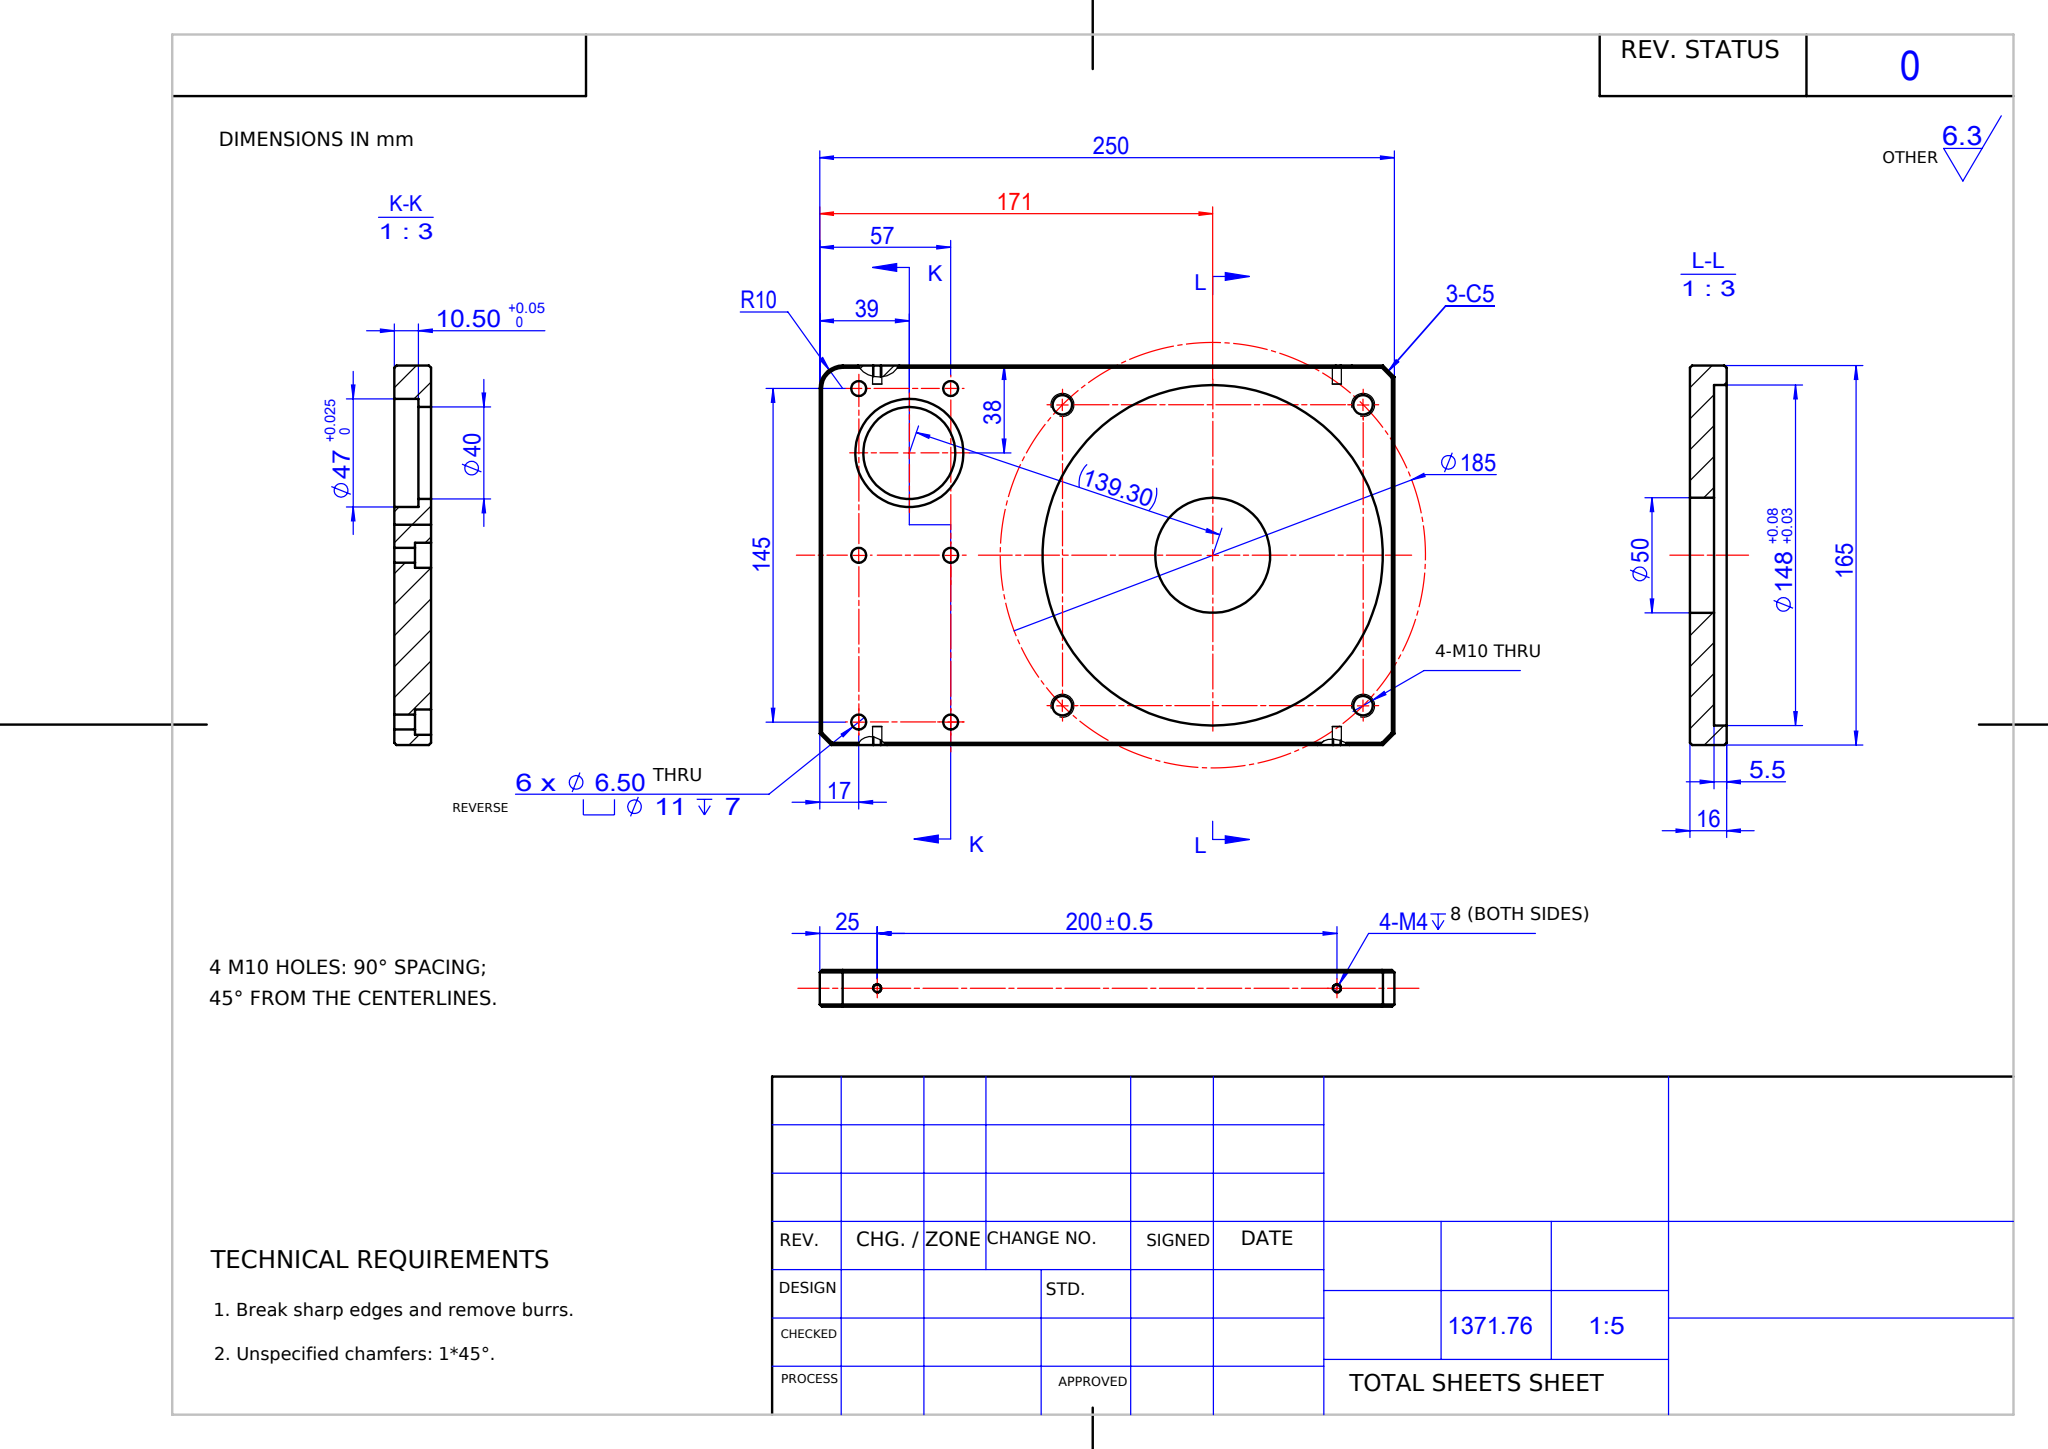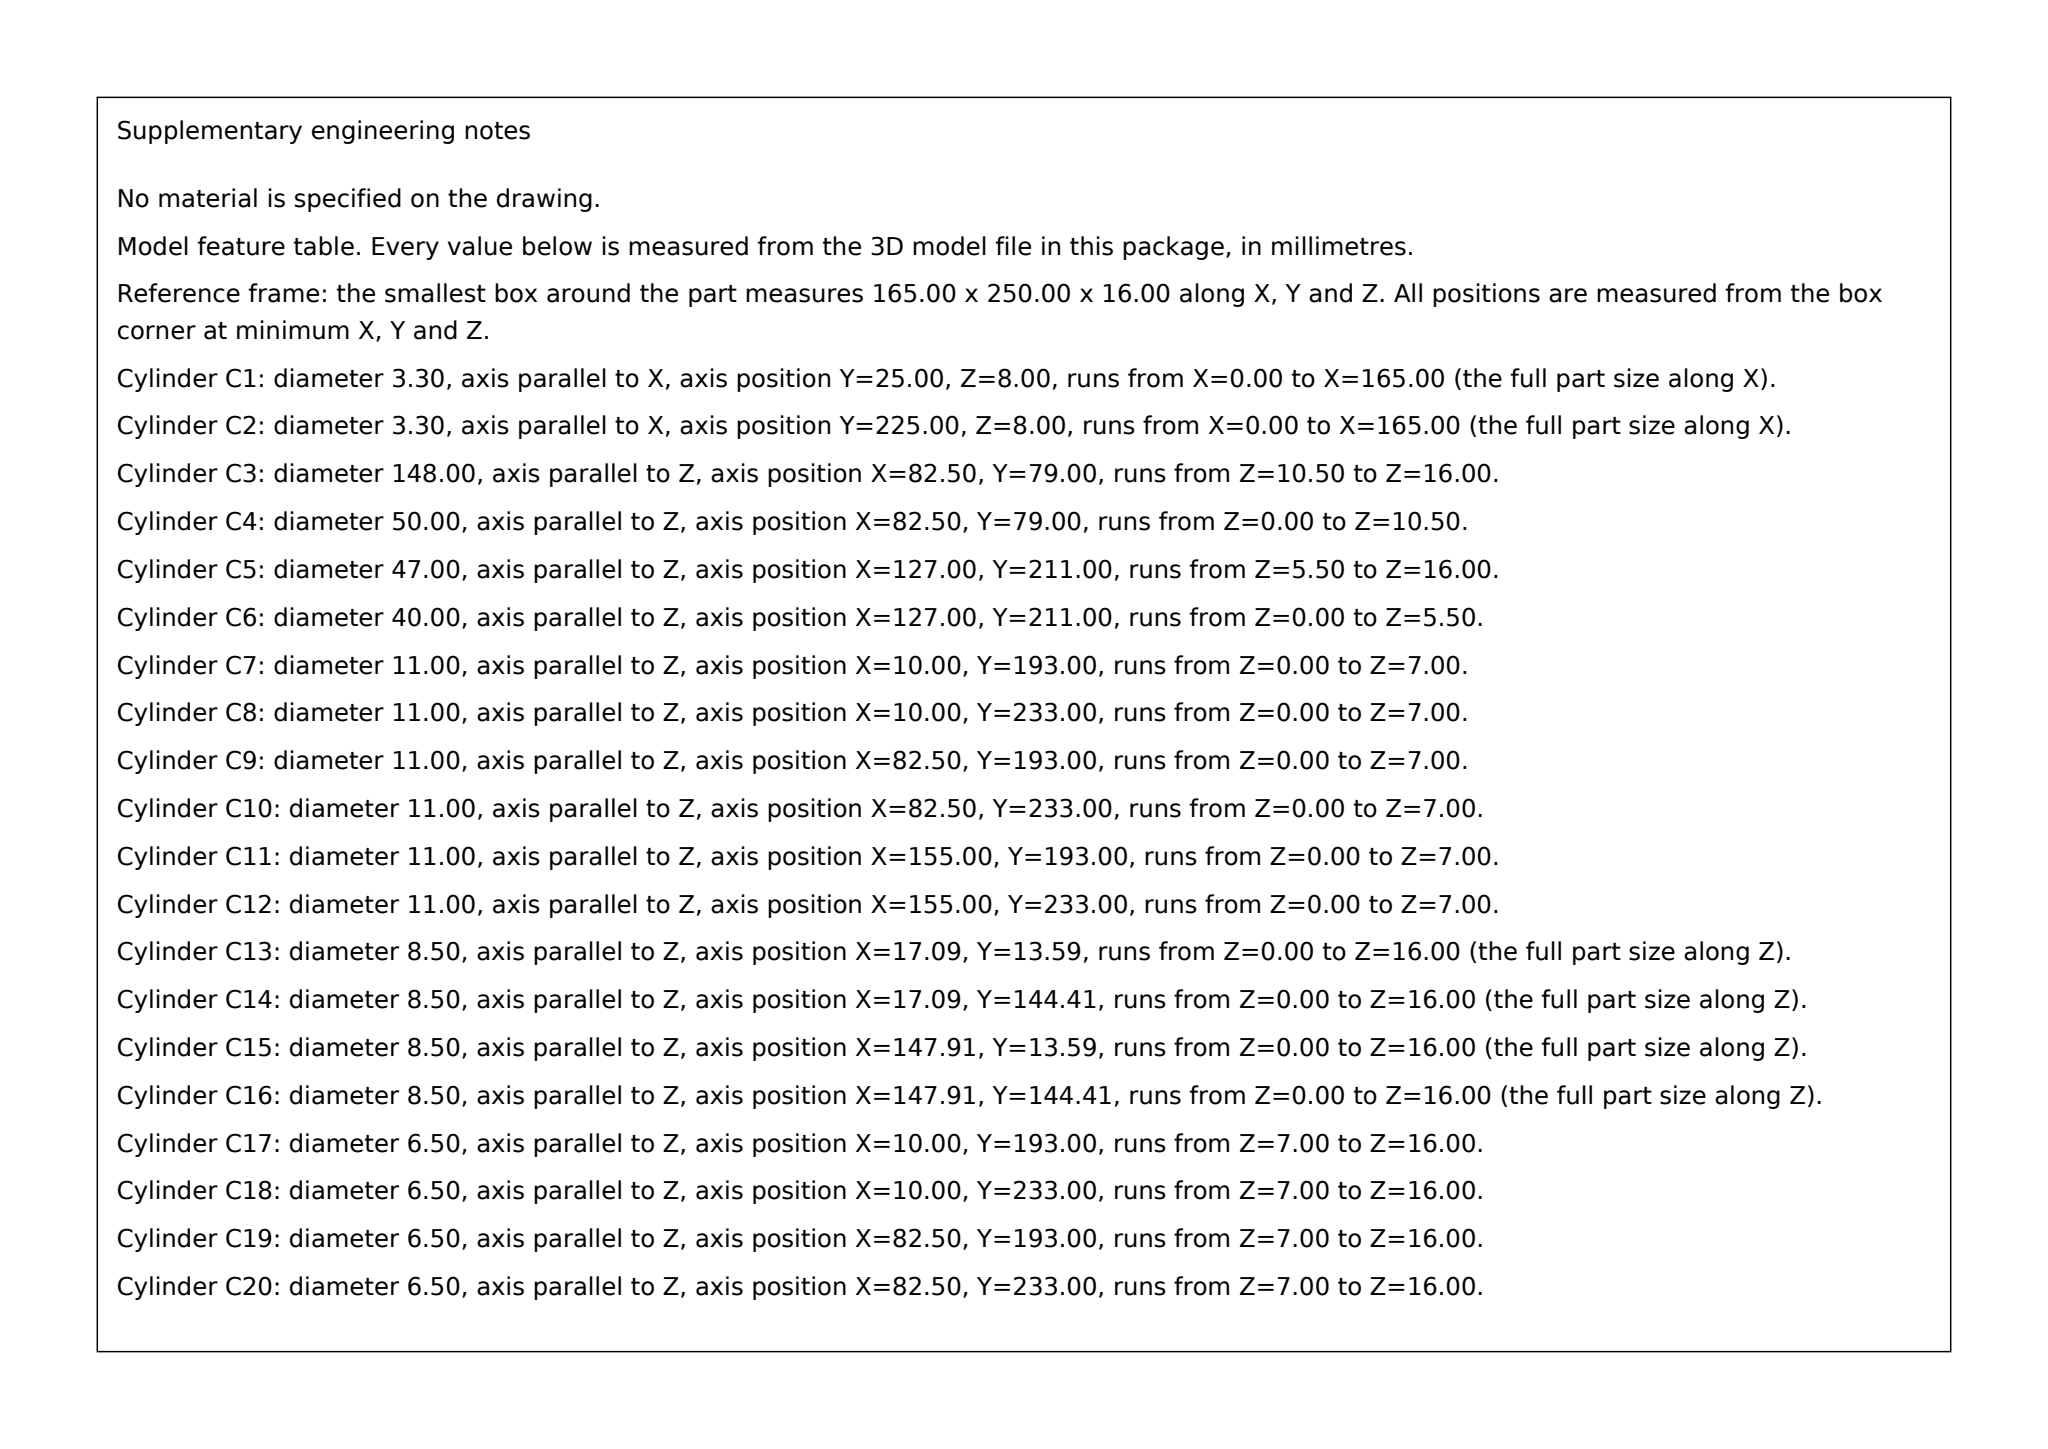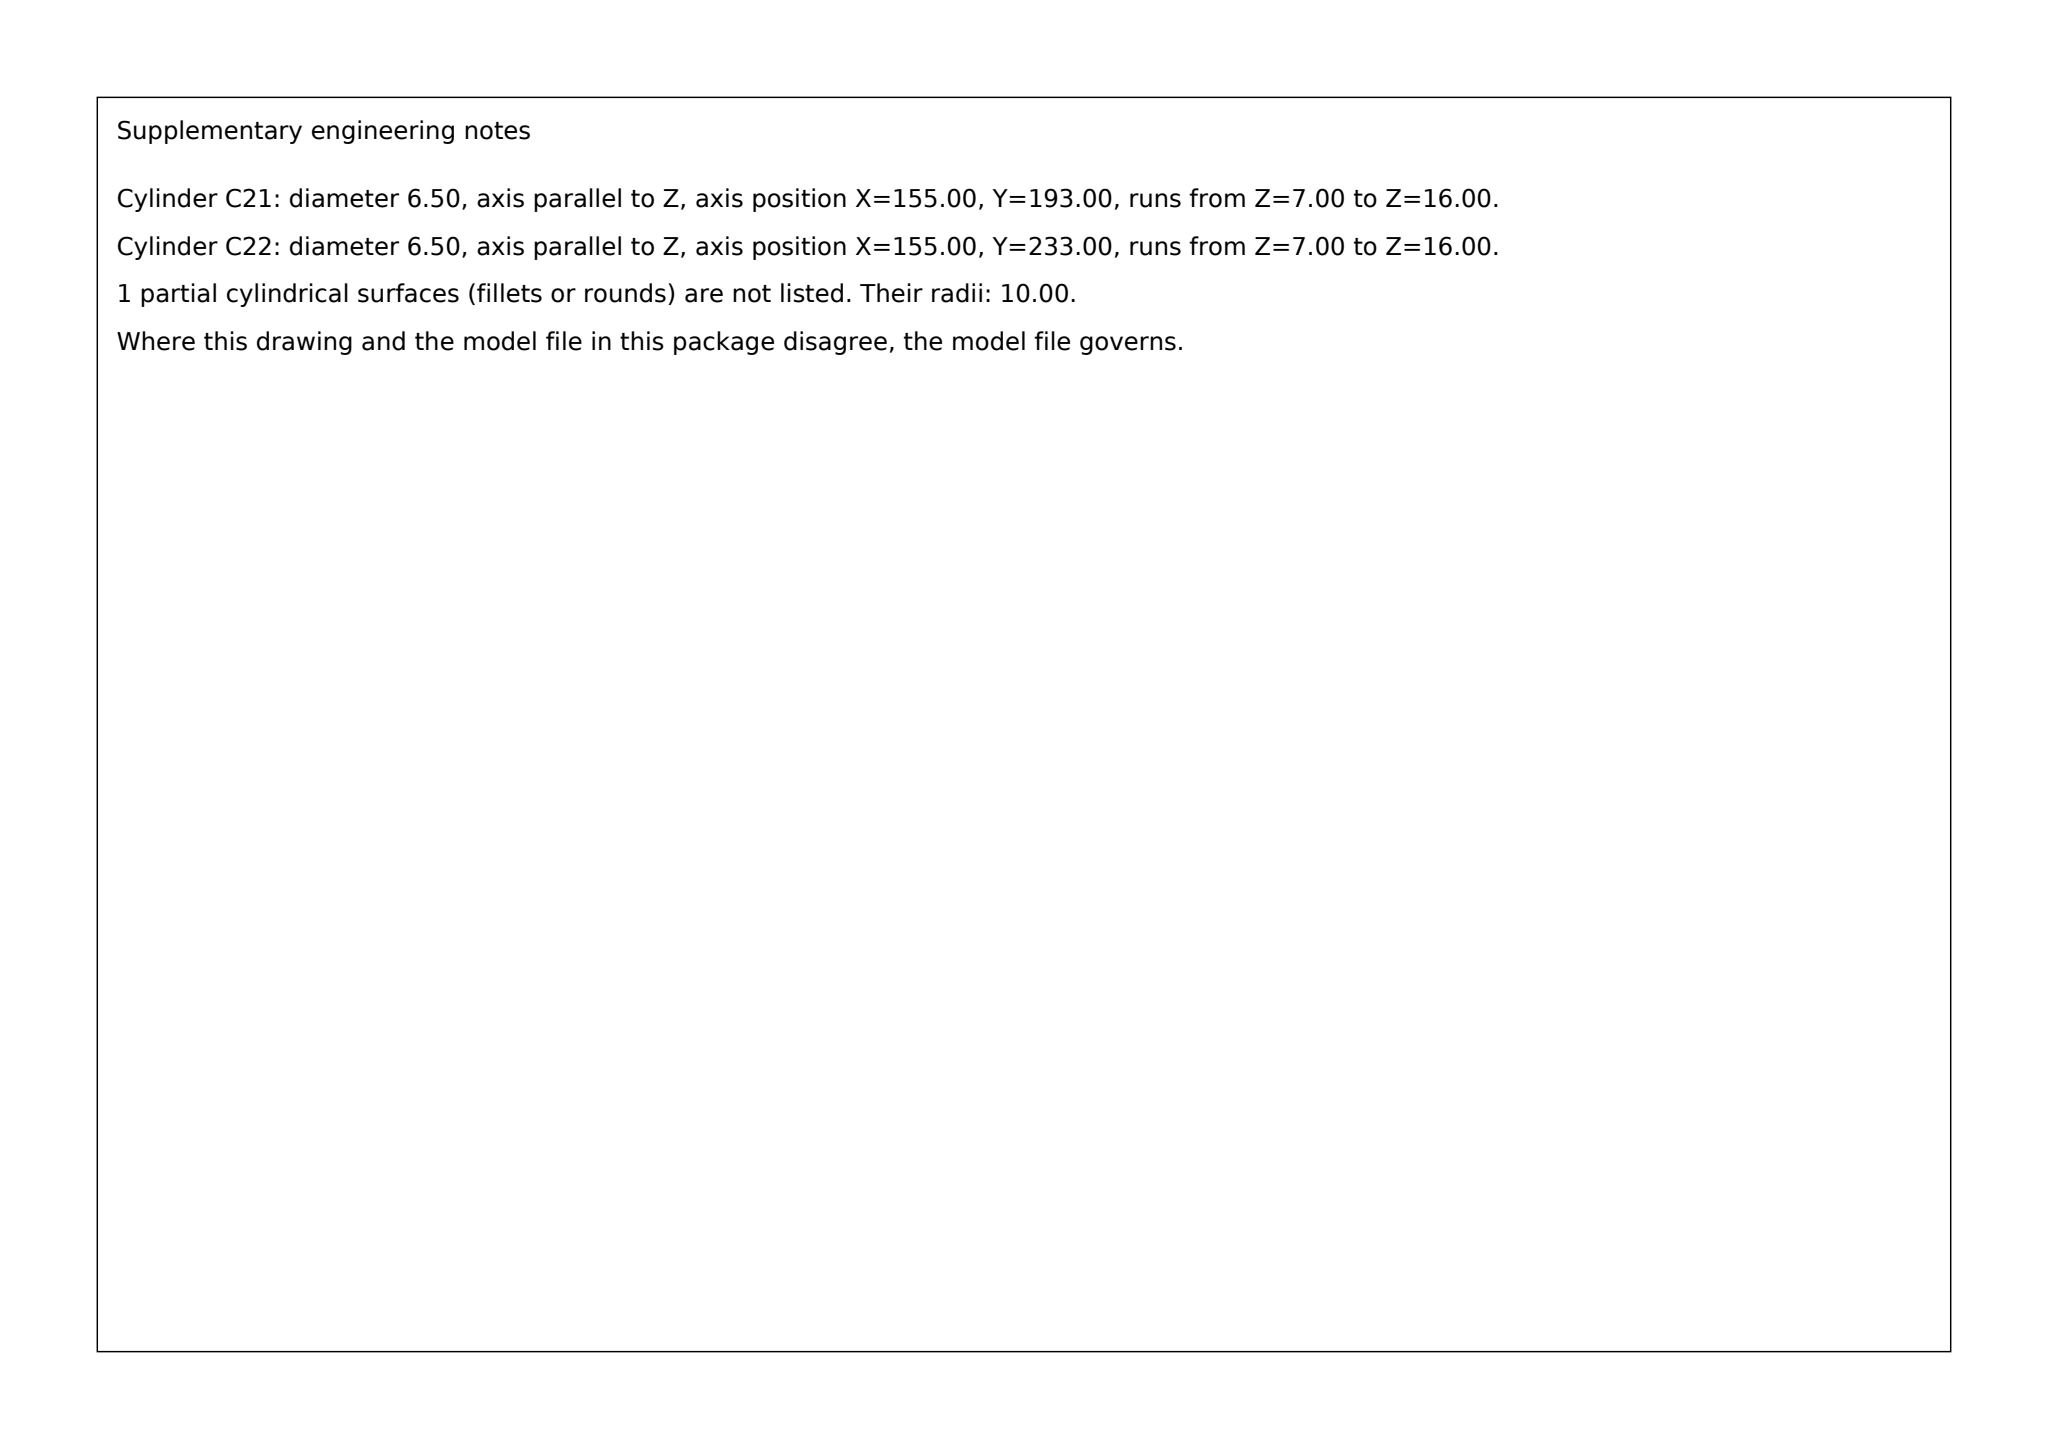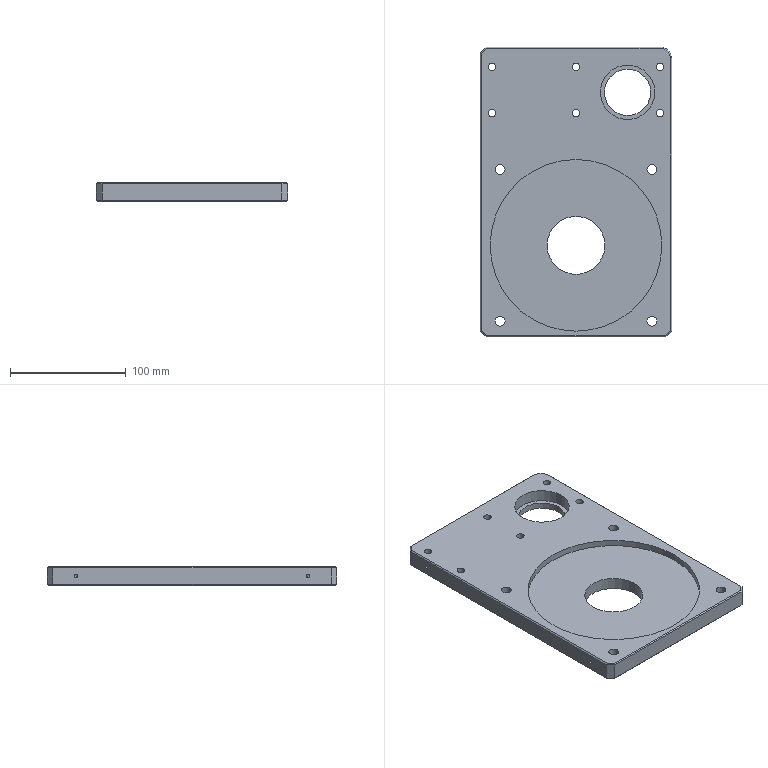Part | SolidWorks | mm | 1 solid | 90 faces | box 165 x 250 x 16 mm | volume 508059 mm3 | cylinder 49 | plane 31 | cone 10 | commonest cylinder face diameters 11 x12 6.5 x12 3.3 x8 8.5 x8 50 x2 148 x2 47 x2 40 x2
build123d program:
from build123d import *

# Parameters (mm, degrees)
SKETCH1_W                                            = 165
SKETCH1_H                                            = 250
BOSS_EXTRUDE1_DEPTH                                  = 8
SKETCH2_R                                            = 20
CUT_EXTRUDE1_DEPTH                                   = 151.623
FILLET1_R                                            = 10
SKETCH3_R                                            = 23.5
CUT_EXTRUDE2_DEPTH                                   = 10.5
SKETCH4_R                                            = 74
CUT_EXTRUDE3_DEPTH                                   = 5.5
SKETCH5_R                                            = 25
CUT_EXTRUDE4_DEPTH                                   = 151.138
M10_TAPPED_HOLE1_D                                   = 8.5
HOLE_SIZE_ACCORDING_TO_THE_TYPE_OF_HEXAG_D           = 6.5
HOLE_SIZE_ACCORDING_TO_THE_TYPE_OF_HEXAG_CBORE_D     = 11
HOLE_SIZE_ACCORDING_TO_THE_TYPE_OF_HEXAG_CBORE_DEPTH = 7
CHAMFER1_SIZE                                        = 5
CHAMFER2_SIZE                                        = 1
M4_TAPPED_HOLE1_AT_2_COUNT                           = 2
M4_TAPPED_HOLE1_AT_2_PITCH                           = 200


with BuildPart() as part:
    # Sketch1 → Boss-Extrude1 (new, symmetric)
    with BuildSketch(Plane.XY):
        Rectangle(SKETCH1_W, SKETCH1_H)
    extrude(amount=BOSS_EXTRUDE1_DEPTH, both=True)

    # Sketch2 → Cut-Extrude1 (cut, through all)
    with BuildSketch(Plane.XY.offset(8)):
        with Locations((44.5, 86)):
            Circle(SKETCH2_R)
    extrude(amount=-CUT_EXTRUDE1_DEPTH, mode=Mode.SUBTRACT)

    # Fillet1
    fillet1_edges = [part.edges().sort_by_distance(p)[0] for p in [
        (82.5, 125, 0),
    ]]
    fillet(fillet1_edges, radius=FILLET1_R)

    # Sketch3 → Cut-Extrude2 (cut)
    with BuildSketch(Plane.XY.offset(8)):
        with Locations((44.5, 86)):
            Circle(SKETCH3_R)
    extrude(amount=-CUT_EXTRUDE2_DEPTH, mode=Mode.SUBTRACT)

    # Sketch4 → Cut-Extrude3 (cut)
    with BuildSketch(Plane.XY.offset(8)):
        with Locations((0, -46)):
            Circle(SKETCH4_R)
    extrude(amount=-CUT_EXTRUDE3_DEPTH, mode=Mode.SUBTRACT)

    # Sketch5 → Cut-Extrude4 (cut, through all)
    with BuildSketch(Plane.XY.offset(2.5)):
        with Locations((0, -46)):
            Circle(SKETCH5_R)
    extrude(amount=-CUT_EXTRUDE4_DEPTH, mode=Mode.SUBTRACT)

    # M10 Tapped Hole1 (through all)
    with Locations(Plane.XY.offset(8)):
        with Locations((-65.407, 19.407), (65.407, 19.407), (65.407, -111.407), (-65.407, -111.407)):
            Hole(M10_TAPPED_HOLE1_D / 2)

    # Hole Size according to the type of Hexag (through all)
    with Locations(Plane(origin=(0, 0, -8), x_dir=(-1, 0, 0), z_dir=(0, 0, -1))):
        with Locations((-72.5, 68), (0, 68), (72.5, 108), (72.5, 68), (0, 108), (-72.5, 108)):
            CounterBoreHole(HOLE_SIZE_ACCORDING_TO_THE_TYPE_OF_HEXAG_D / 2, HOLE_SIZE_ACCORDING_TO_THE_TYPE_OF_HEXAG_CBORE_D / 2, HOLE_SIZE_ACCORDING_TO_THE_TYPE_OF_HEXAG_CBORE_DEPTH)

    # Chamfer1
    chamfer1_edges = [part.edges().sort_by_distance(p)[0] for p in [
        (82.5, -125, 0),
        (-82.5, -125, 0),
        (-82.5, 125, 0),
    ]]
    chamfer(chamfer1_edges, length=CHAMFER1_SIZE)

    # Chamfer2
    chamfer2_edges = [part.edges().sort_by_distance(p)[0] for p in [
        (82.5, -2.5, -8),
        (82.5, -2.5, 8),
        (0, -125, -8),
        (-82.5, 0, -8),
        (-80, 122.5, -8),
        (-80, -122.5, -8),
        (80, -122.5, -8),
        (0, -125, 8),
        (-82.5, 0, 8),
        (-80, 122.5, 8),
        (-80, -122.5, 8),
        (80, -122.5, 8),
        (-2.5, 125, -8),
        (-2.5, 125, 8),
        (79.571, 122.071, -8),
        (79.571, 122.071, 8),
    ]]
    chamfer(chamfer2_edges, length=CHAMFER2_SIZE)

    # Sketch13 → M4 Tapped Hole1 (revolve, cut)
    with BuildSketch(Plane(origin=(82.5, 100, 0), x_dir=(0, 0, -1), z_dir=(0, 1, 0))):
        Polygon((0, 0), (0, 12.491), (1.65, 11.5), (1.65, 0), align=None)
    m4_tapped_hole1 = revolve(axis=Axis((88.85, 100, 0), (-1, 0, 0)), mode=Mode.SUBTRACT)

    # M4 Tapped Hole1 at 2: M4 Tapped Hole1 ×2
    with Locations(*[(0, -i * M4_TAPPED_HOLE1_AT_2_PITCH, 0) for i in range(1, M4_TAPPED_HOLE1_AT_2_COUNT)]):
        add(m4_tapped_hole1, mode=Mode.SUBTRACT)

    # Mirror1: M4 Tapped Hole1 across plane
    add(m4_tapped_hole1.mirror(Plane(origin=(0, 0, 0), x_dir=(0, 0, 1), z_dir=(1, 0, 0))), mode=Mode.SUBTRACT)

    # Mirror1 copy 1 sketch → Mirror1 copy 1 (revolve, cut)
    with BuildSketch(Plane(origin=(-82.5, -100, 0), x_dir=(0, 0, -1), z_dir=(0, 1, 0))):
        Polygon((0, 0), (0, -12.491), (1.65, -11.5), (1.65, 0), align=None)
    revolve(axis=Axis((-88.85, -100, 0), (-1, 0, 0)), mode=Mode.SUBTRACT)


solid = part.part